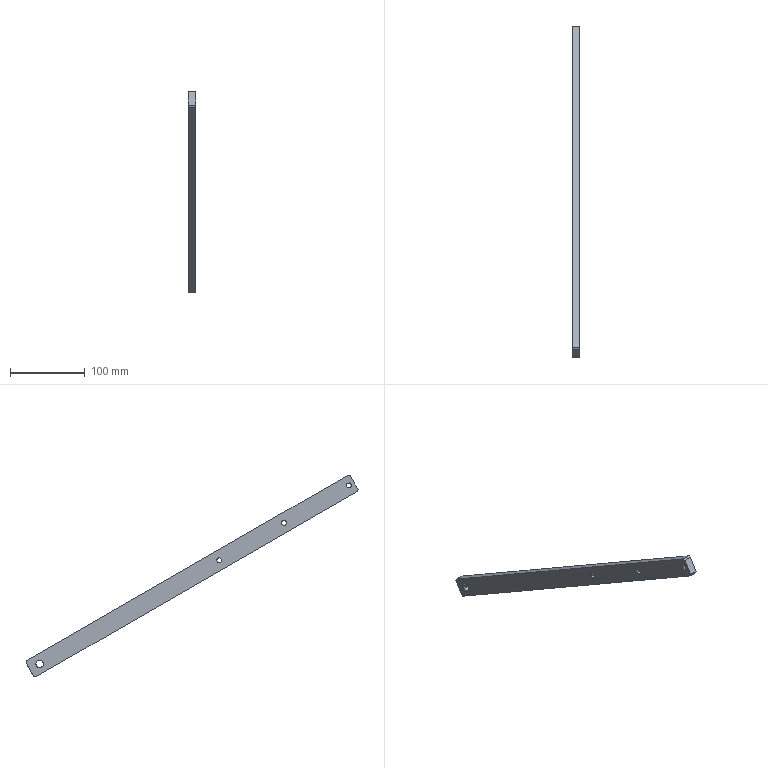Component | SolidWorks | GuideMechanism-1_SwingArm-1_SwingArm.1-1 | 1 solid | 20 faces | box 10 x 443.51 x 269.65 mm | volume 122999 mm3 | cylinder 10 | plane 10 | commonest cylinder face diameters 6.5 x6 4.2 x2 10 x2
build123d program:
from build123d import *

# Parameters (mm, degrees)
SKETCH1_W             = 500
SKETCH1_H             = 25
SKETCH1_R             = 5
BOSS_EXTRUDE1_DEPTH   = 10
M5_TAPPED_HOLE2_D     = 4.2
M5_TAPPED_HOLE2_DEPTH = 15
M5_TAPPED_HOLE2_TIP   = 1.262
CHAMFER1_SIZE         = 2
SKETCH6_R             = 3.25
CUT_EXTRUDE1_DEPTH    = 10


with BuildPart() as part:
    # Sketch1 → Boss-Extrude1 (new body)
    with BuildSketch(Plane.XY):
        Rectangle(SKETCH1_W, SKETCH1_H)
        with Locations((235, 0)):
            Circle(SKETCH1_R, mode=Mode.SUBTRACT)
    extrude(amount=BOSS_EXTRUDE1_DEPTH)

    # M5 Tapped Hole2
    with Locations(Plane(origin=(250, 0, 0), x_dir=(0, 0, -1), z_dir=(1, 0, 0))):
        with Locations((-5, 0)):
            Hole(M5_TAPPED_HOLE2_D / 2, depth=M5_TAPPED_HOLE2_DEPTH)
            with Locations((0, 0, -(M5_TAPPED_HOLE2_DEPTH + M5_TAPPED_HOLE2_TIP / 2))):  # 118° drill point
                Cone(0, M5_TAPPED_HOLE2_D / 2, M5_TAPPED_HOLE2_TIP, mode=Mode.SUBTRACT)

    # Chamfer1
    chamfer1_edges = [part.edges().sort_by_distance(p)[0] for p in [
        (250, -12.5, 5),
        (-250, -12.5, 5),
        (-250, 12.5, 5),
        (250, 12.5, 5),
    ]]
    chamfer(chamfer1_edges, length=CHAMFER1_SIZE)

    # Sketch6 → Cut-Extrude1 (cut)
    with BuildSketch(Plane(origin=(0, 0, 0), x_dir=(-1, 0, 0), z_dir=(0, 0, -1))):
        with Locations((242, 0)):
            Circle(SKETCH6_R)
        with Locations((142, 0)):
            Circle(SKETCH6_R)
        with Locations((42, 0)):
            Circle(SKETCH6_R)
    extrude(amount=-CUT_EXTRUDE1_DEPTH, mode=Mode.SUBTRACT)


solid = part.part

# Placed as in the assembly
solid = solid.moved(Location((-506.772, -772.282, 1514), (60, 90, 0)))
STEP:
#1=COLOUR_RGB('',0.7922,0.8196,0.9333);
#2=FILL_AREA_STYLE_COLOUR('',#1);
#3=FILL_AREA_STYLE('',(#2));
#4=SURFACE_STYLE_FILL_AREA(#3);
#5=SURFACE_SIDE_STYLE('',(#4));
#6=SURFACE_STYLE_USAGE(.BOTH.,#5);
#7=PRESENTATION_STYLE_ASSIGNMENT((#6));
#8=CARTESIAN_POINT('',(-19.952,-35.136,62.338));
#9=VERTEX_POINT('',#8);
#10=CARTESIAN_POINT('',(-19.952,-35.357,62.466));
#11=VERTEX_POINT('',#10);
#12=CARTESIAN_POINT('',(-19.952,-35.246,62.402));
#13=DIRECTION('',(1.,0.,0.));
#14=DIRECTION('',(0.,-0.866,0.5));
#15=AXIS2_PLACEMENT_3D('',#12,#13,#14);
#16=CIRCLE('',#15,0.128);
#17=EDGE_CURVE('',#9,#11,#16,.T.);
#18=ORIENTED_EDGE('',*,*,#17,.F.);
#19=CARTESIAN_POINT('',(-19.558,-35.136,62.338));
#20=VERTEX_POINT('',#19);
#21=CARTESIAN_POINT('',(-19.952,-35.136,62.338));
#22=DIRECTION('',(1.,0.,0.));
#23=VECTOR('',#22,39.37);
#24=LINE('',#21,#23);
#25=EDGE_CURVE('',#9,#20,#24,.T.);
#26=ORIENTED_EDGE('',*,*,#25,.T.);
#27=CARTESIAN_POINT('',(-19.558,-35.357,62.466));
#28=VERTEX_POINT('',#27);
#29=CARTESIAN_POINT('',(-19.558,-35.246,62.402));
#30=DIRECTION('',(1.,0.,0.));
#31=DIRECTION('',(0.,-0.866,0.5));
#32=AXIS2_PLACEMENT_3D('',#29,#30,#31);
#33=CIRCLE('',#32,0.128);
#34=EDGE_CURVE('',#20,#28,#33,.T.);
#35=ORIENTED_EDGE('',*,*,#34,.T.);
#36=CARTESIAN_POINT('',(-19.952,-35.357,62.466));
#37=DIRECTION('',(1.,0.,0.));
#38=VECTOR('',#37,39.37);
#39=LINE('',#36,#38);
#40=EDGE_CURVE('',#11,#28,#39,.T.);
#41=ORIENTED_EDGE('',*,*,#40,.F.);
#42=EDGE_LOOP('',(#18,#26,#35,#41));
#43=FACE_OUTER_BOUND('',#42,.T.);
#44=CARTESIAN_POINT('',(-19.952,-35.246,62.402));
#45=DIRECTION('',(1.,0.,0.));
#46=DIRECTION('',(0.,-0.866,0.5));
#47=AXIS2_PLACEMENT_3D('',#44,#45,#46);
#48=CYLINDRICAL_SURFACE('',#47,0.128);
#49=ADVANCED_FACE('',(#43),#48,.F.);
#50=CARTESIAN_POINT('',(-19.952,-31.726,60.369));
#51=VERTEX_POINT('',#50);
#52=CARTESIAN_POINT('',(-19.952,-31.948,60.497));
#53=VERTEX_POINT('',#52);
#54=CARTESIAN_POINT('',(-19.952,-31.837,60.433));
#55=DIRECTION('',(1.,0.,0.));
#56=DIRECTION('',(0.,-0.866,0.5));
#57=AXIS2_PLACEMENT_3D('',#54,#55,#56);
#58=CIRCLE('',#57,0.128);
#59=EDGE_CURVE('',#51,#53,#58,.T.);
#60=ORIENTED_EDGE('',*,*,#59,.F.);
#61=CARTESIAN_POINT('',(-19.558,-31.726,60.369));
#62=VERTEX_POINT('',#61);
#63=CARTESIAN_POINT('',(-19.952,-31.726,60.369));
#64=DIRECTION('',(1.,0.,0.));
#65=VECTOR('',#64,39.37);
#66=LINE('',#63,#65);
#67=EDGE_CURVE('',#51,#62,#66,.T.);
#68=ORIENTED_EDGE('',*,*,#67,.T.);
#69=CARTESIAN_POINT('',(-19.558,-31.948,60.497));
#70=VERTEX_POINT('',#69);
#71=CARTESIAN_POINT('',(-19.558,-31.837,60.433));
#72=DIRECTION('',(1.,0.,0.));
#73=DIRECTION('',(0.,-0.866,0.5));
#74=AXIS2_PLACEMENT_3D('',#71,#72,#73);
#75=CIRCLE('',#74,0.128);
#76=EDGE_CURVE('',#62,#70,#75,.T.);
#77=ORIENTED_EDGE('',*,*,#76,.T.);
#78=CARTESIAN_POINT('',(-19.952,-31.948,60.497));
#79=DIRECTION('',(1.,0.,0.));
#80=VECTOR('',#79,39.37);
#81=LINE('',#78,#80);
#82=EDGE_CURVE('',#53,#70,#81,.T.);
#83=ORIENTED_EDGE('',*,*,#82,.F.);
#84=EDGE_LOOP('',(#60,#68,#77,#83));
#85=FACE_OUTER_BOUND('',#84,.T.);
#86=CARTESIAN_POINT('',(-19.952,-31.837,60.433));
#87=DIRECTION('',(1.,0.,0.));
#88=DIRECTION('',(0.,-0.866,0.5));
#89=AXIS2_PLACEMENT_3D('',#86,#87,#88);
#90=CYLINDRICAL_SURFACE('',#89,0.128);
#91=ADVANCED_FACE('',(#85),#90,.F.);
#92=CARTESIAN_POINT('',(-19.952,-38.545,64.306));
#93=VERTEX_POINT('',#92);
#94=CARTESIAN_POINT('',(-19.952,-38.767,64.434));
#95=VERTEX_POINT('',#94);
#96=CARTESIAN_POINT('',(-19.952,-38.656,64.37));
#97=DIRECTION('',(1.,0.,0.));
#98=DIRECTION('',(0.,-0.866,0.5));
#99=AXIS2_PLACEMENT_3D('',#96,#97,#98);
#100=CIRCLE('',#99,0.128);
#101=EDGE_CURVE('',#93,#95,#100,.T.);
#102=ORIENTED_EDGE('',*,*,#101,.F.);
#103=CARTESIAN_POINT('',(-19.558,-38.545,64.306));
#104=VERTEX_POINT('',#103);
#105=CARTESIAN_POINT('',(-19.952,-38.545,64.306));
#106=DIRECTION('',(1.,0.,0.));
#107=VECTOR('',#106,39.37);
#108=LINE('',#105,#107);
#109=EDGE_CURVE('',#93,#104,#108,.T.);
#110=ORIENTED_EDGE('',*,*,#109,.T.);
#111=CARTESIAN_POINT('',(-19.558,-38.767,64.434));
#112=VERTEX_POINT('',#111);
#113=CARTESIAN_POINT('',(-19.558,-38.656,64.37));
#114=DIRECTION('',(1.,0.,0.));
#115=DIRECTION('',(0.,-0.866,0.5));
#116=AXIS2_PLACEMENT_3D('',#113,#114,#115);
#117=CIRCLE('',#116,0.128);
#118=EDGE_CURVE('',#104,#112,#117,.T.);
#119=ORIENTED_EDGE('',*,*,#118,.T.);
#120=CARTESIAN_POINT('',(-19.952,-38.767,64.434));
#121=DIRECTION('',(1.,0.,0.));
#122=VECTOR('',#121,39.37);
#123=LINE('',#120,#122);
#124=EDGE_CURVE('',#95,#112,#123,.T.);
#125=ORIENTED_EDGE('',*,*,#124,.F.);
#126=EDGE_LOOP('',(#102,#110,#119,#125));
#127=FACE_OUTER_BOUND('',#126,.T.);
#128=CARTESIAN_POINT('',(-19.952,-38.656,64.37));
#129=DIRECTION('',(1.,0.,0.));
#130=DIRECTION('',(0.,-0.866,0.5));
#131=AXIS2_PLACEMENT_3D('',#128,#129,#130);
#132=CYLINDRICAL_SURFACE('',#131,0.128);
#133=ADVANCED_FACE('',(#127),#132,.F.);
#134=CARTESIAN_POINT('',(-19.672,-22.222,54.882));
#135=VERTEX_POINT('',#134);
#136=CARTESIAN_POINT('',(-19.837,-22.222,54.882));
#137=VERTEX_POINT('',#136);
#138=CARTESIAN_POINT('',(-19.672,-22.222,54.882));
#139=CARTESIAN_POINT('',(-19.672,-22.219,54.887));
#140=CARTESIAN_POINT('',(-19.673,-22.217,54.891));
#141=CARTESIAN_POINT('',(-19.675,-22.212,54.901));
#142=CARTESIAN_POINT('',(-19.676,-22.21,54.906));
#143=CARTESIAN_POINT('',(-19.681,-22.206,54.916));
#144=CARTESIAN_POINT('',(-19.683,-22.205,54.92));
#145=CARTESIAN_POINT('',(-19.689,-22.202,54.929));
#146=CARTESIAN_POINT('',(-19.693,-22.201,54.933));
#147=CARTESIAN_POINT('',(-19.704,-22.199,54.945));
#148=CARTESIAN_POINT('',(-19.713,-22.198,54.951));
#149=CARTESIAN_POINT('',(-19.728,-22.197,54.958));
#150=CARTESIAN_POINT('',(-19.733,-22.197,54.96));
#151=CARTESIAN_POINT('',(-19.744,-22.196,54.962));
#152=CARTESIAN_POINT('',(-19.749,-22.196,54.963));
#153=CARTESIAN_POINT('',(-19.76,-22.196,54.963));
#154=CARTESIAN_POINT('',(-19.766,-22.196,54.962));
#155=CARTESIAN_POINT('',(-19.776,-22.197,54.96));
#156=CARTESIAN_POINT('',(-19.782,-22.197,54.958));
#157=CARTESIAN_POINT('',(-19.792,-22.197,54.953));
#158=CARTESIAN_POINT('',(-19.796,-22.198,54.951));
#159=CARTESIAN_POINT('',(-19.805,-22.199,54.944));
#160=CARTESIAN_POINT('',(-19.81,-22.199,54.941));
#161=CARTESIAN_POINT('',(-19.817,-22.201,54.933));
#162=CARTESIAN_POINT('',(-19.82,-22.202,54.929));
#163=CARTESIAN_POINT('',(-19.826,-22.205,54.92));
#164=CARTESIAN_POINT('',(-19.829,-22.206,54.915));
#165=CARTESIAN_POINT('',(-19.835,-22.212,54.901));
#166=CARTESIAN_POINT('',(-19.837,-22.216,54.891));
#167=CARTESIAN_POINT('',(-19.837,-22.222,54.882));
#168=B_SPLINE_CURVE_WITH_KNOTS('',3,(#138,#139,#140,#141,#142,#143,#144,#145,#146,#147,#148,#149,#150,#151,#152,#153,#154,#155,#156,#157,#158,#159,#160,#161,#162,#163,#164,#165,#166,#167),.UNSPECIFIED.,.F.,.F.,(4,2,2,2,2,2,2,2,2,2,2,2,2,2,4),(0.,0.0004152,0.0008304,0.001246,0.001661,0.002491,0.002907,0.003322,0.003737,0.004152,0.004567,0.004983,0.005398,0.005813,0.006644),.UNSPECIFIED.);
#169=EDGE_CURVE('',#135,#137,#168,.T.);
#170=ORIENTED_EDGE('',*,*,#169,.T.);
#171=CARTESIAN_POINT('',(-19.837,-21.881,54.685));
#172=VERTEX_POINT('',#171);
#173=CARTESIAN_POINT('',(-19.837,-21.881,54.685));
#174=DIRECTION('',(0.,0.866,-0.5));
#175=VECTOR('',#174,39.37);
#176=LINE('',#173,#175);
#177=EDGE_CURVE('',#137,#172,#176,.T.);
#178=ORIENTED_EDGE('',*,*,#177,.T.);
#179=CARTESIAN_POINT('',(-19.672,-21.881,54.685));
#180=VERTEX_POINT('',#179);
#181=CARTESIAN_POINT('',(-19.755,-21.881,54.685));
#182=DIRECTION('',(0.,0.866,-0.5));
#183=DIRECTION('',(1.,0.,0.));
#184=AXIS2_PLACEMENT_3D('',#181,#182,#183);
#185=CIRCLE('',#184,0.08268);
#186=EDGE_CURVE('',#172,#180,#185,.T.);
#187=ORIENTED_EDGE('',*,*,#186,.T.);
#188=CARTESIAN_POINT('',(-19.672,-21.881,54.685));
#189=DIRECTION('',(0.,0.866,-0.5));
#190=VECTOR('',#189,39.37);
#191=LINE('',#188,#190);
#192=EDGE_CURVE('',#135,#180,#191,.T.);
#193=ORIENTED_EDGE('',*,*,#192,.F.);
#194=EDGE_LOOP('',(#170,#178,#187,#193));
#195=FACE_OUTER_BOUND('',#194,.T.);
#196=CARTESIAN_POINT('',(-19.755,-21.881,54.685));
#197=DIRECTION('',(0.,0.866,-0.5));
#198=DIRECTION('',(1.,0.,0.));
#199=AXIS2_PLACEMENT_3D('',#196,#197,#198);
#200=CYLINDRICAL_SURFACE('',#199,0.08268);
#201=ADVANCED_FACE('',(#195),#200,.F.);
#202=CARTESIAN_POINT('',(-19.952,-22.563,55.079));
#203=VERTEX_POINT('',#202);
#204=CARTESIAN_POINT('',(-19.952,-22.222,54.882));
#205=VERTEX_POINT('',#204);
#206=CARTESIAN_POINT('',(-19.952,-22.392,54.98));
#207=DIRECTION('',(-1.,-0.,-0.));
#208=DIRECTION('',(0.,0.866,-0.5));
#209=AXIS2_PLACEMENT_3D('',#206,#207,#208);
#210=CIRCLE('',#209,0.1969);
#211=EDGE_CURVE('',#203,#205,#210,.T.);
#212=ORIENTED_EDGE('',*,*,#211,.T.);
#213=CARTESIAN_POINT('',(-19.952,-22.222,54.882));
#214=DIRECTION('',(1.,0.,0.));
#215=VECTOR('',#214,39.37);
#216=LINE('',#213,#215);
#217=EDGE_CURVE('',#205,#137,#216,.T.);
#218=ORIENTED_EDGE('',*,*,#217,.T.);
#219=ORIENTED_EDGE('',*,*,#169,.F.);
#220=CARTESIAN_POINT('',(-19.558,-22.222,54.882));
#221=VERTEX_POINT('',#220);
#222=CARTESIAN_POINT('',(-19.952,-22.222,54.882));
#223=DIRECTION('',(1.,0.,0.));
#224=VECTOR('',#223,39.37);
#225=LINE('',#222,#224);
#226=EDGE_CURVE('',#135,#221,#225,.T.);
#227=ORIENTED_EDGE('',*,*,#226,.T.);
#228=CARTESIAN_POINT('',(-19.558,-22.563,55.079));
#229=VERTEX_POINT('',#228);
#230=CARTESIAN_POINT('',(-19.558,-22.392,54.98));
#231=DIRECTION('',(-1.,-0.,-0.));
#232=DIRECTION('',(0.,0.866,-0.5));
#233=AXIS2_PLACEMENT_3D('',#230,#231,#232);
#234=CIRCLE('',#233,0.1969);
#235=EDGE_CURVE('',#229,#221,#234,.T.);
#236=ORIENTED_EDGE('',*,*,#235,.F.);
#237=CARTESIAN_POINT('',(-19.952,-22.563,55.079));
#238=DIRECTION('',(1.,0.,0.));
#239=VECTOR('',#238,39.37);
#240=LINE('',#237,#239);
#241=EDGE_CURVE('',#203,#229,#240,.T.);
#242=ORIENTED_EDGE('',*,*,#241,.F.);
#243=EDGE_LOOP('',(#212,#218,#219,#227,#236,#242));
#244=FACE_OUTER_BOUND('',#243,.T.);
#245=CARTESIAN_POINT('',(-19.952,-22.392,54.98));
#246=DIRECTION('',(1.,0.,0.));
#247=DIRECTION('',(0.,-0.866,0.5));
#248=AXIS2_PLACEMENT_3D('',#245,#246,#247);
#249=CYLINDRICAL_SURFACE('',#248,0.1969);
#250=ADVANCED_FACE('',(#244),#249,.F.);
#251=CARTESIAN_POINT('',(-19.952,-35.246,62.402));
#252=DIRECTION('',(1.,0.,0.));
#253=DIRECTION('',(0.,-0.866,0.5));
#254=AXIS2_PLACEMENT_3D('',#251,#252,#253);
#255=CIRCLE('',#254,0.128);
#256=EDGE_CURVE('',#11,#9,#255,.T.);
#257=ORIENTED_EDGE('',*,*,#256,.T.);
#258=ORIENTED_EDGE('',*,*,#17,.T.);
#259=EDGE_LOOP('',(#257,#258));
#260=FACE_BOUND('',#259,.T.);
#261=CARTESIAN_POINT('',(-19.952,-31.837,60.433));
#262=DIRECTION('',(1.,0.,0.));
#263=DIRECTION('',(0.,-0.866,0.5));
#264=AXIS2_PLACEMENT_3D('',#261,#262,#263);
#265=CIRCLE('',#264,0.128);
#266=EDGE_CURVE('',#53,#51,#265,.T.);
#267=ORIENTED_EDGE('',*,*,#266,.T.);
#268=ORIENTED_EDGE('',*,*,#59,.T.);
#269=EDGE_LOOP('',(#267,#268));
#270=FACE_BOUND('',#269,.T.);
#271=CARTESIAN_POINT('',(-19.952,-38.656,64.37));
#272=DIRECTION('',(1.,0.,0.));
#273=DIRECTION('',(0.,-0.866,0.5));
#274=AXIS2_PLACEMENT_3D('',#271,#272,#273);
#275=CIRCLE('',#274,0.128);
#276=EDGE_CURVE('',#95,#93,#275,.T.);
#277=ORIENTED_EDGE('',*,*,#276,.T.);
#278=ORIENTED_EDGE('',*,*,#101,.T.);
#279=EDGE_LOOP('',(#277,#278));
#280=FACE_BOUND('',#279,.T.);
#281=CARTESIAN_POINT('',(-19.952,-38.614,64.914));
#282=VERTEX_POINT('',#281);
#283=CARTESIAN_POINT('',(-19.952,-21.703,55.151));
#284=VERTEX_POINT('',#283);
#285=CARTESIAN_POINT('',(-19.952,-38.683,64.954));
#286=DIRECTION('',(0.,0.866,-0.5));
#287=VECTOR('',#286,39.37);
#288=LINE('',#285,#287);
#289=EDGE_CURVE('',#282,#284,#288,.T.);
#290=ORIENTED_EDGE('',*,*,#289,.T.);
#291=CARTESIAN_POINT('',(-19.952,-21.674,55.043));
#292=VERTEX_POINT('',#291);
#293=CARTESIAN_POINT('',(-19.952,-23.4,61.483));
#294=DIRECTION('',(0.,0.2588,-0.9659));
#295=VECTOR('',#294,39.37);
#296=LINE('',#293,#295);
#297=EDGE_CURVE('',#284,#292,#296,.T.);
#298=ORIENTED_EDGE('',*,*,#297,.T.);
#299=CARTESIAN_POINT('',(-19.952,-22.088,54.327));
#300=VERTEX_POINT('',#299);
#301=CARTESIAN_POINT('',(-19.952,-22.127,54.259));
#302=DIRECTION('',(0.,-0.5,-0.866));
#303=VECTOR('',#302,39.37);
#304=LINE('',#301,#303);
#305=EDGE_CURVE('',#292,#300,#304,.T.);
#306=ORIENTED_EDGE('',*,*,#305,.T.);
#307=CARTESIAN_POINT('',(-19.952,-22.195,54.298));
#308=VERTEX_POINT('',#307);
#309=CARTESIAN_POINT('',(-19.952,-28.528,52.601));
#310=DIRECTION('',(0.,-0.9659,-0.2588));
#311=VECTOR('',#310,39.37);
#312=LINE('',#309,#311);
#313=EDGE_CURVE('',#300,#308,#312,.T.);
#314=ORIENTED_EDGE('',*,*,#313,.T.);
#315=CARTESIAN_POINT('',(-19.952,-39.107,64.062));
#316=VERTEX_POINT('',#315);
#317=CARTESIAN_POINT('',(-19.952,-39.175,64.101));
#318=DIRECTION('',(-0.,-0.866,0.5));
#319=VECTOR('',#318,39.37);
#320=LINE('',#317,#319);
#321=EDGE_CURVE('',#308,#316,#320,.T.);
#322=ORIENTED_EDGE('',*,*,#321,.T.);
#323=CARTESIAN_POINT('',(-19.952,-39.135,64.17));
#324=VERTEX_POINT('',#323);
#325=CARTESIAN_POINT('',(-19.952,-37.41,57.729));
#326=DIRECTION('',(-0.,-0.2588,0.9659));
#327=VECTOR('',#326,39.37);
#328=LINE('',#325,#327);
#329=EDGE_CURVE('',#316,#324,#328,.T.);
#330=ORIENTED_EDGE('',*,*,#329,.T.);
#331=CARTESIAN_POINT('',(-19.952,-38.722,64.886));
#332=VERTEX_POINT('',#331);
#333=CARTESIAN_POINT('',(-19.952,-39.175,64.101));
#334=DIRECTION('',(-0.,0.5,0.866));
#335=VECTOR('',#334,39.37);
#336=LINE('',#333,#335);
#337=EDGE_CURVE('',#324,#332,#336,.T.);
#338=ORIENTED_EDGE('',*,*,#337,.T.);
#339=CARTESIAN_POINT('',(-19.952,-32.282,66.611));
#340=DIRECTION('',(-0.,0.9659,0.2588));
#341=VECTOR('',#340,39.37);
#342=LINE('',#339,#341);
#343=EDGE_CURVE('',#332,#282,#342,.T.);
#344=ORIENTED_EDGE('',*,*,#343,.T.);
#345=EDGE_LOOP('',(#290,#298,#306,#314,#322,#330,#338,#344));
#346=FACE_OUTER_BOUND('',#345,.T.);
#347=ORIENTED_EDGE('',*,*,#211,.F.);
#348=CARTESIAN_POINT('',(-19.952,-22.392,54.98));
#349=DIRECTION('',(-1.,-0.,-0.));
#350=DIRECTION('',(0.,0.866,-0.5));
#351=AXIS2_PLACEMENT_3D('',#348,#349,#350);
#352=CIRCLE('',#351,0.1969);
#353=EDGE_CURVE('',#205,#203,#352,.T.);
#354=ORIENTED_EDGE('',*,*,#353,.F.);
#355=EDGE_LOOP('',(#347,#354));
#356=FACE_BOUND('',#355,.T.);
#357=CARTESIAN_POINT('',(-19.952,-30.405,59.606));
#358=DIRECTION('',(-1.,-0.,-0.));
#359=DIRECTION('',(0.,0.866,-0.5));
#360=AXIS2_PLACEMENT_3D('',#357,#358,#359);
#361=PLANE('',#360);
#362=ADVANCED_FACE('',(#260,#270,#280,#346,#356),#361,.T.);
#363=CARTESIAN_POINT('',(-19.558,-35.246,62.402));
#364=DIRECTION('',(1.,0.,0.));
#365=DIRECTION('',(0.,-0.866,0.5));
#366=AXIS2_PLACEMENT_3D('',#363,#364,#365);
#367=CIRCLE('',#366,0.128);
#368=EDGE_CURVE('',#28,#20,#367,.T.);
#369=ORIENTED_EDGE('',*,*,#368,.F.);
#370=ORIENTED_EDGE('',*,*,#34,.F.);
#371=EDGE_LOOP('',(#369,#370));
#372=FACE_BOUND('',#371,.T.);
#373=CARTESIAN_POINT('',(-19.558,-31.837,60.433));
#374=DIRECTION('',(1.,0.,0.));
#375=DIRECTION('',(0.,-0.866,0.5));
#376=AXIS2_PLACEMENT_3D('',#373,#374,#375);
#377=CIRCLE('',#376,0.128);
#378=EDGE_CURVE('',#70,#62,#377,.T.);
#379=ORIENTED_EDGE('',*,*,#378,.F.);
#380=ORIENTED_EDGE('',*,*,#76,.F.);
#381=EDGE_LOOP('',(#379,#380));
#382=FACE_BOUND('',#381,.T.);
#383=CARTESIAN_POINT('',(-19.558,-38.656,64.37));
#384=DIRECTION('',(1.,0.,0.));
#385=DIRECTION('',(0.,-0.866,0.5));
#386=AXIS2_PLACEMENT_3D('',#383,#384,#385);
#387=CIRCLE('',#386,0.128);
#388=EDGE_CURVE('',#112,#104,#387,.T.);
#389=ORIENTED_EDGE('',*,*,#388,.F.);
#390=ORIENTED_EDGE('',*,*,#118,.F.);
#391=EDGE_LOOP('',(#389,#390));
#392=FACE_BOUND('',#391,.T.);
#393=CARTESIAN_POINT('',(-19.558,-21.674,55.043));
#394=VERTEX_POINT('',#393);
#395=CARTESIAN_POINT('',(-19.558,-22.088,54.327));
#396=VERTEX_POINT('',#395);
#397=CARTESIAN_POINT('',(-19.558,-22.127,54.259));
#398=DIRECTION('',(0.,-0.5,-0.866));
#399=VECTOR('',#398,39.37);
#400=LINE('',#397,#399);
#401=EDGE_CURVE('',#394,#396,#400,.T.);
#402=ORIENTED_EDGE('',*,*,#401,.F.);
#403=CARTESIAN_POINT('',(-19.558,-21.703,55.151));
#404=VERTEX_POINT('',#403);
#405=CARTESIAN_POINT('',(-19.558,-21.674,55.043));
#406=DIRECTION('',(-0.,-0.2588,0.9659));
#407=VECTOR('',#406,39.37);
#408=LINE('',#405,#407);
#409=EDGE_CURVE('',#394,#404,#408,.T.);
#410=ORIENTED_EDGE('',*,*,#409,.T.);
#411=CARTESIAN_POINT('',(-19.558,-38.614,64.914));
#412=VERTEX_POINT('',#411);
#413=CARTESIAN_POINT('',(-19.558,-38.683,64.954));
#414=DIRECTION('',(0.,0.866,-0.5));
#415=VECTOR('',#414,39.37);
#416=LINE('',#413,#415);
#417=EDGE_CURVE('',#412,#404,#416,.T.);
#418=ORIENTED_EDGE('',*,*,#417,.F.);
#419=CARTESIAN_POINT('',(-19.558,-38.722,64.886));
#420=VERTEX_POINT('',#419);
#421=CARTESIAN_POINT('',(-19.558,-38.614,64.914));
#422=DIRECTION('',(0.,-0.9659,-0.2588));
#423=VECTOR('',#422,39.37);
#424=LINE('',#421,#423);
#425=EDGE_CURVE('',#412,#420,#424,.T.);
#426=ORIENTED_EDGE('',*,*,#425,.T.);
#427=CARTESIAN_POINT('',(-19.558,-39.135,64.17));
#428=VERTEX_POINT('',#427);
#429=CARTESIAN_POINT('',(-19.558,-39.175,64.101));
#430=DIRECTION('',(-0.,0.5,0.866));
#431=VECTOR('',#430,39.37);
#432=LINE('',#429,#431);
#433=EDGE_CURVE('',#428,#420,#432,.T.);
#434=ORIENTED_EDGE('',*,*,#433,.F.);
#435=CARTESIAN_POINT('',(-19.558,-39.107,64.062));
#436=VERTEX_POINT('',#435);
#437=CARTESIAN_POINT('',(-19.558,-39.135,64.17));
#438=DIRECTION('',(0.,0.2588,-0.9659));
#439=VECTOR('',#438,39.37);
#440=LINE('',#437,#439);
#441=EDGE_CURVE('',#428,#436,#440,.T.);
#442=ORIENTED_EDGE('',*,*,#441,.T.);
#443=CARTESIAN_POINT('',(-19.558,-22.195,54.298));
#444=VERTEX_POINT('',#443);
#445=CARTESIAN_POINT('',(-19.558,-39.175,64.101));
#446=DIRECTION('',(-0.,-0.866,0.5));
#447=VECTOR('',#446,39.37);
#448=LINE('',#445,#447);
#449=EDGE_CURVE('',#444,#436,#448,.T.);
#450=ORIENTED_EDGE('',*,*,#449,.F.);
#451=CARTESIAN_POINT('',(-19.558,-22.195,54.298));
#452=DIRECTION('',(-0.,0.9659,0.2588));
#453=VECTOR('',#452,39.37);
#454=LINE('',#451,#453);
#455=EDGE_CURVE('',#444,#396,#454,.T.);
#456=ORIENTED_EDGE('',*,*,#455,.T.);
#457=EDGE_LOOP('',(#402,#410,#418,#426,#434,#442,#450,#456));
#458=FACE_OUTER_BOUND('',#457,.T.);
#459=ORIENTED_EDGE('',*,*,#235,.T.);
#460=CARTESIAN_POINT('',(-19.558,-22.392,54.98));
#461=DIRECTION('',(-1.,-0.,-0.));
#462=DIRECTION('',(0.,0.866,-0.5));
#463=AXIS2_PLACEMENT_3D('',#460,#461,#462);
#464=CIRCLE('',#463,0.1969);
#465=EDGE_CURVE('',#221,#229,#464,.T.);
#466=ORIENTED_EDGE('',*,*,#465,.T.);
#467=EDGE_LOOP('',(#459,#466));
#468=FACE_BOUND('',#467,.T.);
#469=CARTESIAN_POINT('',(-19.558,-30.405,59.606));
#470=DIRECTION('',(-1.,-0.,-0.));
#471=DIRECTION('',(0.,0.866,-0.5));
#472=AXIS2_PLACEMENT_3D('',#469,#470,#471);
#473=PLANE('',#472);
#474=ADVANCED_FACE('',(#372,#382,#392,#458,#468),#473,.F.);
#475=CARTESIAN_POINT('',(-19.755,-21.881,54.685));
#476=DIRECTION('',(0.,0.866,-0.5));
#477=DIRECTION('',(1.,0.,0.));
#478=AXIS2_PLACEMENT_3D('',#475,#476,#477);
#479=CIRCLE('',#478,0.08268);
#480=EDGE_CURVE('',#180,#172,#479,.T.);
#481=ORIENTED_EDGE('',*,*,#480,.F.);
#482=ORIENTED_EDGE('',*,*,#186,.F.);
#483=EDGE_LOOP('',(#481,#482));
#484=FACE_BOUND('',#483,.T.);
#485=ORIENTED_EDGE('',*,*,#305,.F.);
#486=CARTESIAN_POINT('',(-19.952,-21.674,55.043));
#487=DIRECTION('',(1.,0.,0.));
#488=VECTOR('',#487,39.37);
#489=LINE('',#486,#488);
#490=EDGE_CURVE('',#292,#394,#489,.T.);
#491=ORIENTED_EDGE('',*,*,#490,.T.);
#492=ORIENTED_EDGE('',*,*,#401,.T.);
#493=CARTESIAN_POINT('',(-19.952,-22.088,54.327));
#494=DIRECTION('',(-1.,-0.,-0.));
#495=VECTOR('',#494,39.37);
#496=LINE('',#493,#495);
#497=EDGE_CURVE('',#396,#300,#496,.T.);
#498=ORIENTED_EDGE('',*,*,#497,.T.);
#499=EDGE_LOOP('',(#485,#491,#492,#498));
#500=FACE_OUTER_BOUND('',#499,.T.);
#501=CARTESIAN_POINT('',(-19.952,-22.127,54.259));
#502=DIRECTION('',(-0.,-0.866,0.5));
#503=DIRECTION('',(-1.,-0.,-0.));
#504=AXIS2_PLACEMENT_3D('',#501,#502,#503);
#505=PLANE('',#504);
#506=ADVANCED_FACE('',(#484,#500),#505,.F.);
#507=ORIENTED_EDGE('',*,*,#321,.F.);
#508=CARTESIAN_POINT('',(-19.952,-22.195,54.298));
#509=DIRECTION('',(1.,0.,0.));
#510=VECTOR('',#509,39.37);
#511=LINE('',#508,#510);
#512=EDGE_CURVE('',#308,#444,#511,.T.);
#513=ORIENTED_EDGE('',*,*,#512,.T.);
#514=ORIENTED_EDGE('',*,*,#449,.T.);
#515=CARTESIAN_POINT('',(-19.952,-39.107,64.062));
#516=DIRECTION('',(-1.,-0.,-0.));
#517=VECTOR('',#516,39.37);
#518=LINE('',#515,#517);
#519=EDGE_CURVE('',#436,#316,#518,.T.);
#520=ORIENTED_EDGE('',*,*,#519,.T.);
#521=EDGE_LOOP('',(#507,#513,#514,#520));
#522=FACE_OUTER_BOUND('',#521,.T.);
#523=CARTESIAN_POINT('',(-19.952,-39.175,64.101));
#524=DIRECTION('',(-0.,0.5,0.866));
#525=DIRECTION('',(1.,0.,0.));
#526=AXIS2_PLACEMENT_3D('',#523,#524,#525);
#527=PLANE('',#526);
#528=ADVANCED_FACE('',(#522),#527,.F.);
#529=ORIENTED_EDGE('',*,*,#433,.T.);
#530=CARTESIAN_POINT('',(-19.952,-38.722,64.886));
#531=DIRECTION('',(-1.,-0.,-0.));
#532=VECTOR('',#531,39.37);
#533=LINE('',#530,#532);
#534=EDGE_CURVE('',#420,#332,#533,.T.);
#535=ORIENTED_EDGE('',*,*,#534,.T.);
#536=ORIENTED_EDGE('',*,*,#337,.F.);
#537=CARTESIAN_POINT('',(-19.952,-39.135,64.17));
#538=DIRECTION('',(1.,0.,0.));
#539=VECTOR('',#538,39.37);
#540=LINE('',#537,#539);
#541=EDGE_CURVE('',#324,#428,#540,.T.);
#542=ORIENTED_EDGE('',*,*,#541,.T.);
#543=EDGE_LOOP('',(#529,#535,#536,#542));
#544=FACE_OUTER_BOUND('',#543,.T.);
#545=CARTESIAN_POINT('',(-19.952,-39.175,64.101));
#546=DIRECTION('',(0.,0.866,-0.5));
#547=DIRECTION('',(1.,0.,0.));
#548=AXIS2_PLACEMENT_3D('',#545,#546,#547);
#549=PLANE('',#548);
#550=ADVANCED_FACE('',(#544),#549,.F.);
#551=ORIENTED_EDGE('',*,*,#417,.T.);
#552=CARTESIAN_POINT('',(-19.952,-21.703,55.151));
#553=DIRECTION('',(-1.,-0.,-0.));
#554=VECTOR('',#553,39.37);
#555=LINE('',#552,#554);
#556=EDGE_CURVE('',#404,#284,#555,.T.);
#557=ORIENTED_EDGE('',*,*,#556,.T.);
#558=ORIENTED_EDGE('',*,*,#289,.F.);
#559=CARTESIAN_POINT('',(-19.952,-38.614,64.914));
#560=DIRECTION('',(1.,0.,0.));
#561=VECTOR('',#560,39.37);
#562=LINE('',#559,#561);
#563=EDGE_CURVE('',#282,#412,#562,.T.);
#564=ORIENTED_EDGE('',*,*,#563,.T.);
#565=EDGE_LOOP('',(#551,#557,#558,#564));
#566=FACE_OUTER_BOUND('',#565,.T.);
#567=CARTESIAN_POINT('',(-19.952,-38.683,64.954));
#568=DIRECTION('',(0.,-0.5,-0.866));
#569=DIRECTION('',(-1.,-0.,-0.));
#570=AXIS2_PLACEMENT_3D('',#567,#568,#569);
#571=PLANE('',#570);
#572=ADVANCED_FACE('',(#566),#571,.F.);
#573=ORIENTED_EDGE('',*,*,#217,.F.);
#574=ORIENTED_EDGE('',*,*,#353,.T.);
#575=ORIENTED_EDGE('',*,*,#241,.T.);
#576=ORIENTED_EDGE('',*,*,#465,.F.);
#577=ORIENTED_EDGE('',*,*,#226,.F.);
#578=CARTESIAN_POINT('',(-19.837,-22.222,54.882));
#579=CARTESIAN_POINT('',(-19.837,-22.225,54.877));
#580=CARTESIAN_POINT('',(-19.837,-22.228,54.873));
#581=CARTESIAN_POINT('',(-19.835,-22.234,54.864));
#582=CARTESIAN_POINT('',(-19.833,-22.237,54.86));
#583=CARTESIAN_POINT('',(-19.829,-22.243,54.852));
#584=CARTESIAN_POINT('',(-19.826,-22.247,54.848));
#585=CARTESIAN_POINT('',(-19.82,-22.253,54.841));
#586=CARTESIAN_POINT('',(-19.817,-22.256,54.838));
#587=CARTESIAN_POINT('',(-19.809,-22.262,54.833));
#588=CARTESIAN_POINT('',(-19.805,-22.264,54.831));
#589=CARTESIAN_POINT('',(-19.796,-22.269,54.827));
#590=CARTESIAN_POINT('',(-19.792,-22.272,54.825));
#591=CARTESIAN_POINT('',(-19.782,-22.275,54.822));
#592=CARTESIAN_POINT('',(-19.776,-22.277,54.821));
#593=CARTESIAN_POINT('',(-19.766,-22.278,54.82));
#594=CARTESIAN_POINT('',(-19.76,-22.279,54.819));
#595=CARTESIAN_POINT('',(-19.744,-22.279,54.819));
#596=CARTESIAN_POINT('',(-19.733,-22.277,54.821));
#597=CARTESIAN_POINT('',(-19.718,-22.272,54.825));
#598=CARTESIAN_POINT('',(-19.713,-22.269,54.827));
#599=CARTESIAN_POINT('',(-19.704,-22.264,54.831));
#600=CARTESIAN_POINT('',(-19.7,-22.262,54.833));
#601=CARTESIAN_POINT('',(-19.693,-22.256,54.838));
#602=CARTESIAN_POINT('',(-19.689,-22.253,54.841));
#603=CARTESIAN_POINT('',(-19.683,-22.247,54.848));
#604=CARTESIAN_POINT('',(-19.681,-22.243,54.852));
#605=CARTESIAN_POINT('',(-19.676,-22.237,54.86));
#606=CARTESIAN_POINT('',(-19.675,-22.234,54.864));
#607=CARTESIAN_POINT('',(-19.673,-22.228,54.872));
#608=CARTESIAN_POINT('',(-19.672,-22.225,54.877));
#609=CARTESIAN_POINT('',(-19.672,-22.222,54.882));
#610=B_SPLINE_CURVE_WITH_KNOTS('',3,(#578,#579,#580,#581,#582,#583,#584,#585,#586,#587,#588,#589,#590,#591,#592,#593,#594,#595,#596,#597,#598,#599,#600,#601,#602,#603,#604,#605,#606,#607,#608,#609),.UNSPECIFIED.,.F.,.F.,(4,2,2,2,2,2,2,2,2,2,2,2,2,2,2,4),(0.006644,0.007058,0.007473,0.007888,0.008303,0.008718,0.009133,0.009548,0.009963,0.01079,0.01121,0.01162,0.01204,0.01245,0.01287,0.01328),.UNSPECIFIED.);
#611=EDGE_CURVE('',#137,#135,#610,.T.);
#612=ORIENTED_EDGE('',*,*,#611,.F.);
#613=EDGE_LOOP('',(#573,#574,#575,#576,#577,#612));
#614=FACE_OUTER_BOUND('',#613,.T.);
#615=CARTESIAN_POINT('',(-19.952,-22.392,54.98));
#616=DIRECTION('',(1.,0.,0.));
#617=DIRECTION('',(0.,-0.866,0.5));
#618=AXIS2_PLACEMENT_3D('',#615,#616,#617);
#619=CYLINDRICAL_SURFACE('',#618,0.1969);
#620=ADVANCED_FACE('',(#614),#619,.F.);
#621=ORIENTED_EDGE('',*,*,#177,.F.);
#622=ORIENTED_EDGE('',*,*,#611,.T.);
#623=ORIENTED_EDGE('',*,*,#192,.T.);
#624=ORIENTED_EDGE('',*,*,#480,.T.);
#625=EDGE_LOOP('',(#621,#622,#623,#624));
#626=FACE_OUTER_BOUND('',#625,.T.);
#627=CARTESIAN_POINT('',(-19.755,-21.881,54.685));
#628=DIRECTION('',(0.,0.866,-0.5));
#629=DIRECTION('',(1.,0.,0.));
#630=AXIS2_PLACEMENT_3D('',#627,#628,#629);
#631=CYLINDRICAL_SURFACE('',#630,0.08268);
#632=ADVANCED_FACE('',(#626),#631,.F.);
#633=ORIENTED_EDGE('',*,*,#297,.F.);
#634=ORIENTED_EDGE('',*,*,#556,.F.);
#635=ORIENTED_EDGE('',*,*,#409,.F.);
#636=ORIENTED_EDGE('',*,*,#490,.F.);
#637=EDGE_LOOP('',(#633,#634,#635,#636));
#638=FACE_OUTER_BOUND('',#637,.T.);
#639=CARTESIAN_POINT('',(-19.952,-21.674,55.043));
#640=DIRECTION('',(0.,-0.9659,-0.2588));
#641=DIRECTION('',(1.,0.,0.));
#642=AXIS2_PLACEMENT_3D('',#639,#640,#641);
#643=PLANE('',#642);
#644=ADVANCED_FACE('',(#638),#643,.F.);
#645=ORIENTED_EDGE('',*,*,#313,.F.);
#646=ORIENTED_EDGE('',*,*,#497,.F.);
#647=ORIENTED_EDGE('',*,*,#455,.F.);
#648=ORIENTED_EDGE('',*,*,#512,.F.);
#649=EDGE_LOOP('',(#645,#646,#647,#648));
#650=FACE_OUTER_BOUND('',#649,.T.);
#651=CARTESIAN_POINT('',(-19.952,-22.195,54.298));
#652=DIRECTION('',(-0.,-0.2588,0.9659));
#653=DIRECTION('',(1.,0.,0.));
#654=AXIS2_PLACEMENT_3D('',#651,#652,#653);
#655=PLANE('',#654);
#656=ADVANCED_FACE('',(#650),#655,.F.);
#657=ORIENTED_EDGE('',*,*,#343,.F.);
#658=ORIENTED_EDGE('',*,*,#534,.F.);
#659=ORIENTED_EDGE('',*,*,#425,.F.);
#660=ORIENTED_EDGE('',*,*,#563,.F.);
#661=EDGE_LOOP('',(#657,#658,#659,#660));
#662=FACE_OUTER_BOUND('',#661,.T.);
#663=CARTESIAN_POINT('',(-19.952,-38.614,64.914));
#664=DIRECTION('',(0.,0.2588,-0.9659));
#665=DIRECTION('',(1.,0.,0.));
#666=AXIS2_PLACEMENT_3D('',#663,#664,#665);
#667=PLANE('',#666);
#668=ADVANCED_FACE('',(#662),#667,.F.);
#669=ORIENTED_EDGE('',*,*,#329,.F.);
#670=ORIENTED_EDGE('',*,*,#519,.F.);
#671=ORIENTED_EDGE('',*,*,#441,.F.);
#672=ORIENTED_EDGE('',*,*,#541,.F.);
#673=EDGE_LOOP('',(#669,#670,#671,#672));
#674=FACE_OUTER_BOUND('',#673,.T.);
#675=CARTESIAN_POINT('',(-19.952,-39.135,64.17));
#676=DIRECTION('',(-0.,0.9659,0.2588));
#677=DIRECTION('',(1.,0.,0.));
#678=AXIS2_PLACEMENT_3D('',#675,#676,#677);
#679=PLANE('',#678);
#680=ADVANCED_FACE('',(#674),#679,.F.);
#681=ORIENTED_EDGE('',*,*,#109,.F.);
#682=ORIENTED_EDGE('',*,*,#276,.F.);
#683=ORIENTED_EDGE('',*,*,#124,.T.);
#684=ORIENTED_EDGE('',*,*,#388,.T.);
#685=EDGE_LOOP('',(#681,#682,#683,#684));
#686=FACE_OUTER_BOUND('',#685,.T.);
#687=CARTESIAN_POINT('',(-19.952,-38.656,64.37));
#688=DIRECTION('',(1.,0.,0.));
#689=DIRECTION('',(0.,-0.866,0.5));
#690=AXIS2_PLACEMENT_3D('',#687,#688,#689);
#691=CYLINDRICAL_SURFACE('',#690,0.128);
#692=ADVANCED_FACE('',(#686),#691,.F.);
#693=ORIENTED_EDGE('',*,*,#67,.F.);
#694=ORIENTED_EDGE('',*,*,#266,.F.);
#695=ORIENTED_EDGE('',*,*,#82,.T.);
#696=ORIENTED_EDGE('',*,*,#378,.T.);
#697=EDGE_LOOP('',(#693,#694,#695,#696));
#698=FACE_OUTER_BOUND('',#697,.T.);
#699=CARTESIAN_POINT('',(-19.952,-31.837,60.433));
#700=DIRECTION('',(1.,0.,0.));
#701=DIRECTION('',(0.,-0.866,0.5));
#702=AXIS2_PLACEMENT_3D('',#699,#700,#701);
#703=CYLINDRICAL_SURFACE('',#702,0.128);
#704=ADVANCED_FACE('',(#698),#703,.F.);
#705=ORIENTED_EDGE('',*,*,#25,.F.);
#706=ORIENTED_EDGE('',*,*,#256,.F.);
#707=ORIENTED_EDGE('',*,*,#40,.T.);
#708=ORIENTED_EDGE('',*,*,#368,.T.);
#709=EDGE_LOOP('',(#705,#706,#707,#708));
#710=FACE_OUTER_BOUND('',#709,.T.);
#711=CARTESIAN_POINT('',(-19.952,-35.246,62.402));
#712=DIRECTION('',(1.,0.,0.));
#713=DIRECTION('',(0.,-0.866,0.5));
#714=AXIS2_PLACEMENT_3D('',#711,#712,#713);
#715=CYLINDRICAL_SURFACE('',#714,0.128);
#716=ADVANCED_FACE('',(#710),#715,.F.);
#717=CLOSED_SHELL('',(#49,#91,#133,#201,#250,#362,#474,#506,#528,#550,#572,#620,#632,#644,#656,#668,#680,#692,#704,#716));
#718=MANIFOLD_SOLID_BREP('',#717);
#719=STYLED_ITEM('',(#7),#718);
#720=(LENGTH_UNIT()NAMED_UNIT(*)SI_UNIT($,.METRE.));
#721=LENGTH_MEASURE_WITH_UNIT(LENGTH_MEASURE(0.0254),#720);
#722=DIMENSIONAL_EXPONENTS(1.,0.,0.,0.,0.,0.,0.);
#723=(CONVERSION_BASED_UNIT('',#721)LENGTH_UNIT()NAMED_UNIT(#722));
#724=UNCERTAINTY_MEASURE_WITH_UNIT(LENGTH_MEASURE(0.00001),#723,'','');
#725=(NAMED_UNIT(*)PLANE_ANGLE_UNIT()SI_UNIT($,.RADIAN.));
#726=(NAMED_UNIT(*)SI_UNIT($,.STERADIAN.)SOLID_ANGLE_UNIT());
#727=(GEOMETRIC_REPRESENTATION_CONTEXT(3)GLOBAL_UNCERTAINTY_ASSIGNED_CONTEXT((#724))GLOBAL_UNIT_ASSIGNED_CONTEXT((#723,#725,#726))REPRESENTATION_CONTEXT('',''));
#728=MECHANICAL_DESIGN_GEOMETRIC_PRESENTATION_REPRESENTATION('',(#719),#727);
#729=CARTESIAN_POINT('',(0.,0.,0.));
#730=DIRECTION('',(0.,0.,1.));
#731=DIRECTION('',(1.,0.,0.));
#732=AXIS2_PLACEMENT_3D('',#729,#730,#731);
#733=(LENGTH_UNIT()NAMED_UNIT(*)SI_UNIT($,.METRE.));
#734=LENGTH_MEASURE_WITH_UNIT(LENGTH_MEASURE(0.0254),#733);
#735=DIMENSIONAL_EXPONENTS(1.,0.,0.,0.,0.,0.,0.);
#736=(CONVERSION_BASED_UNIT('',#734)LENGTH_UNIT()NAMED_UNIT(#735));
#737=UNCERTAINTY_MEASURE_WITH_UNIT(LENGTH_MEASURE(0.00001),#736,'','');
#738=(NAMED_UNIT(*)PLANE_ANGLE_UNIT()SI_UNIT($,.RADIAN.));
#739=(NAMED_UNIT(*)SI_UNIT($,.STERADIAN.)SOLID_ANGLE_UNIT());
#740=(GEOMETRIC_REPRESENTATION_CONTEXT(3)GLOBAL_UNCERTAINTY_ASSIGNED_CONTEXT((#737))GLOBAL_UNIT_ASSIGNED_CONTEXT((#736,#738,#739))REPRESENTATION_CONTEXT('',''));
#741=ADVANCED_BREP_SHAPE_REPRESENTATION('',(#718,#732),#740);
#742=PRESENTATION_LAYER_ASSIGNMENT('','',(#719));